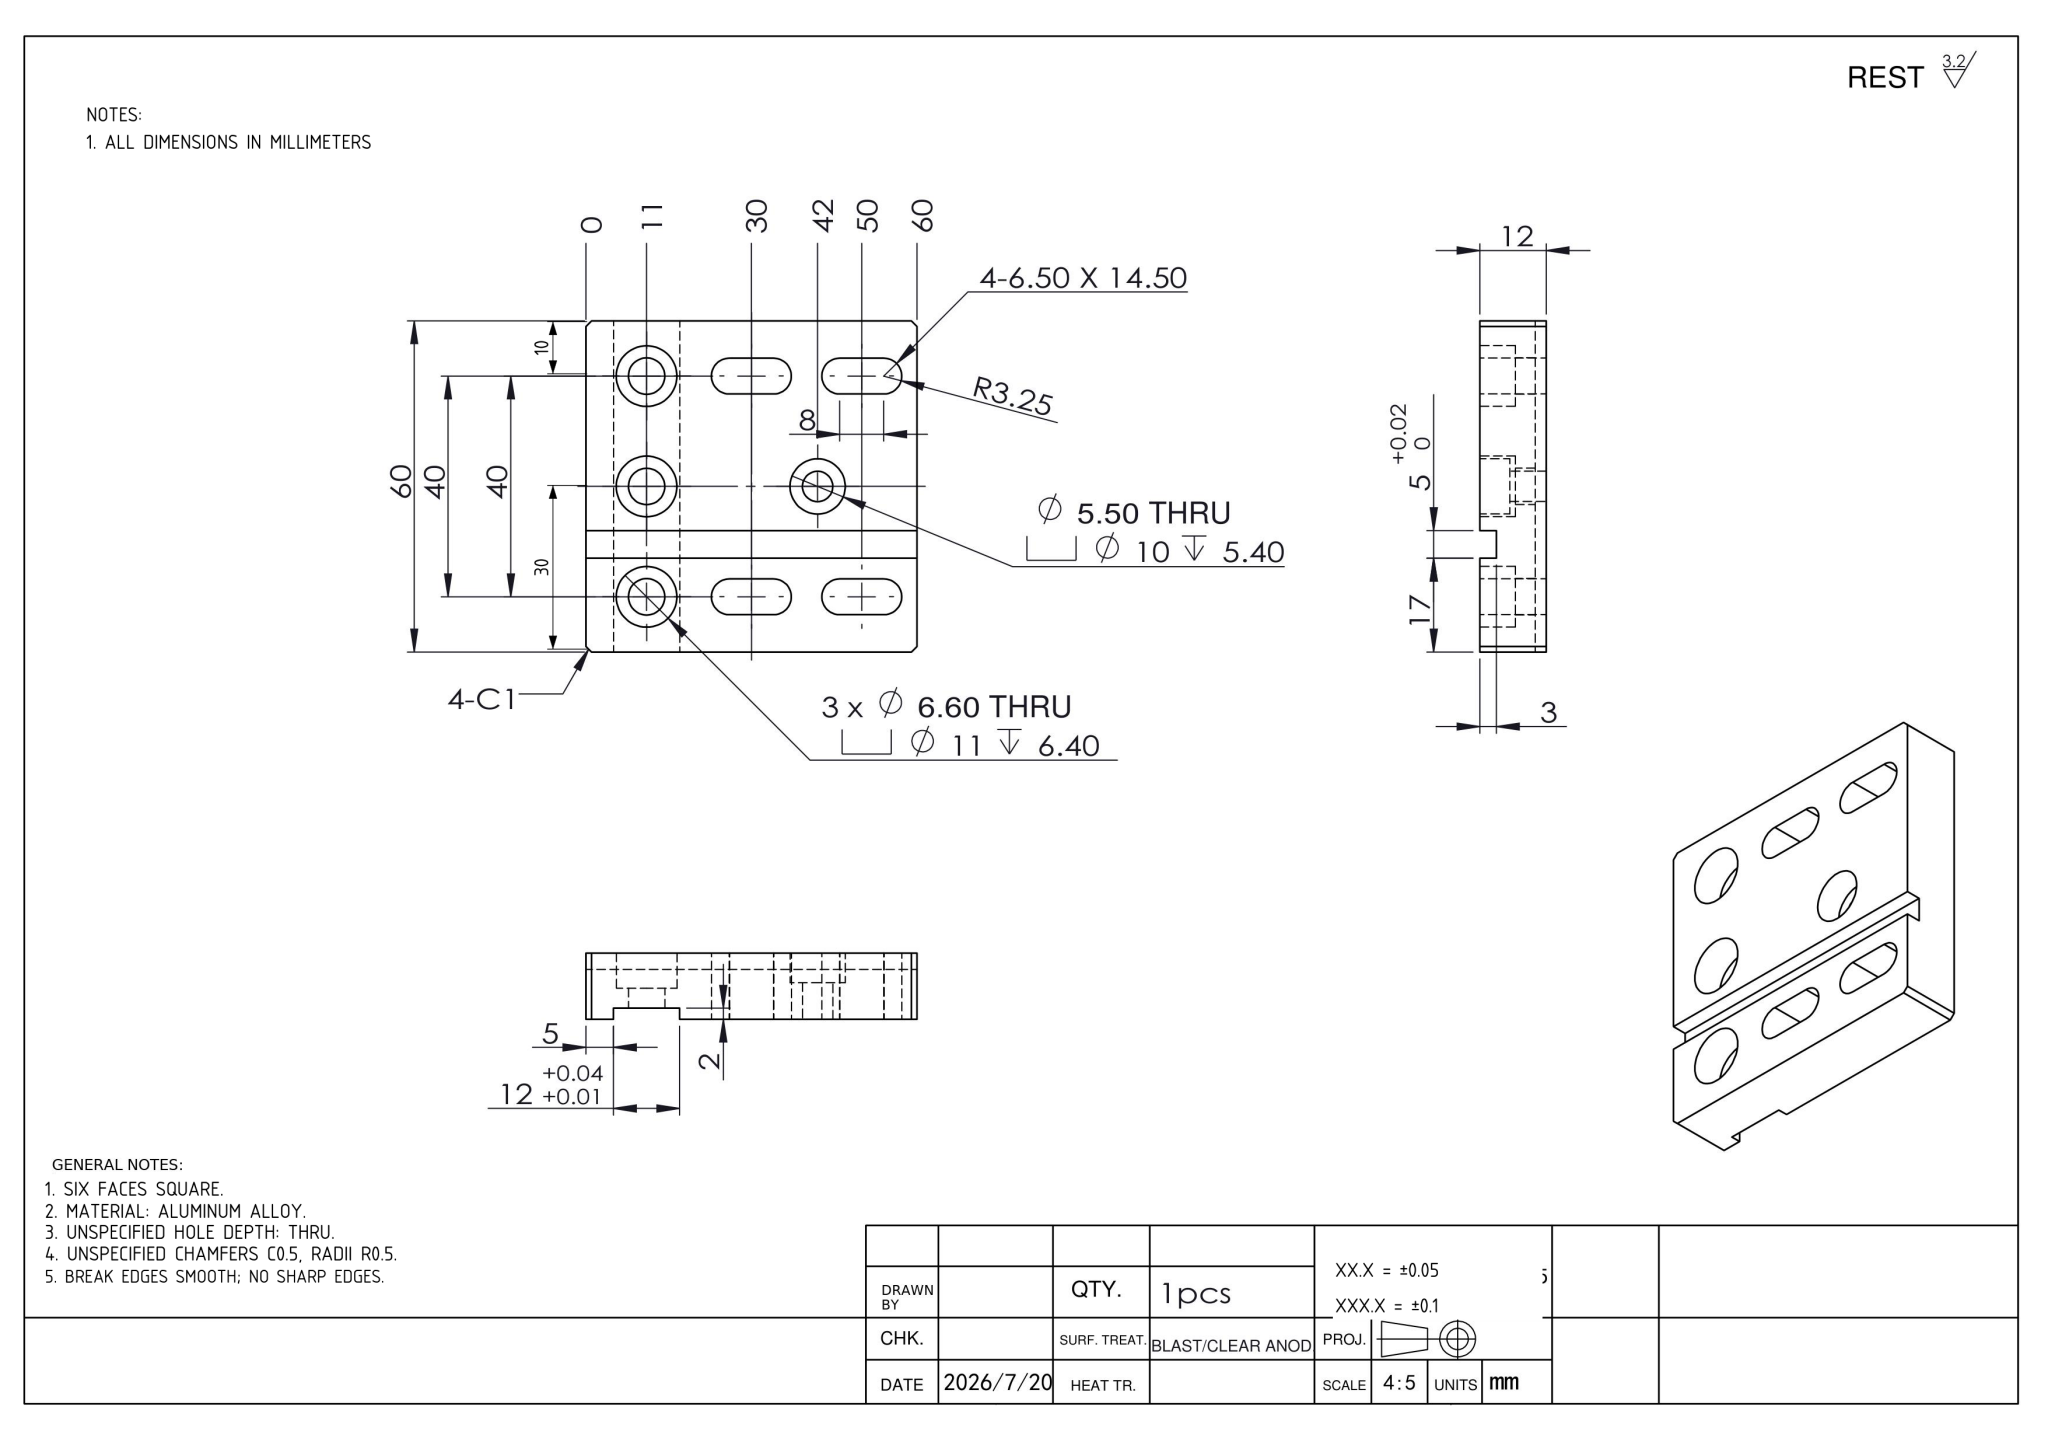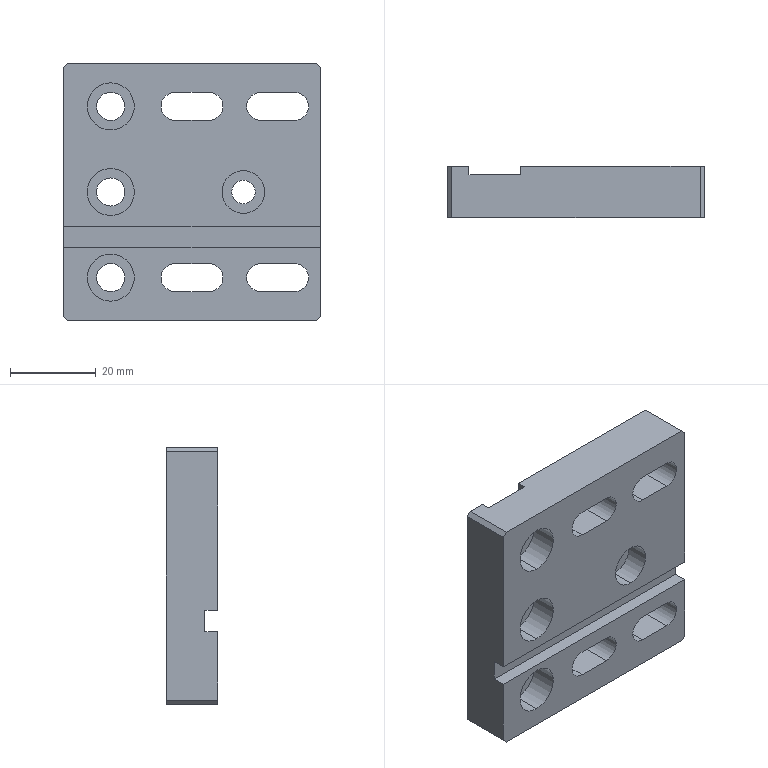Part | NX | mm | 1 solid | 54 faces | box 60 x 12 x 60 mm | volume 33972 mm3 | plane 30 | cylinder 24 | commonest cylinder face diameters 6.5 x8 11 x6 6.6 x6 10 x2 5.5 x2